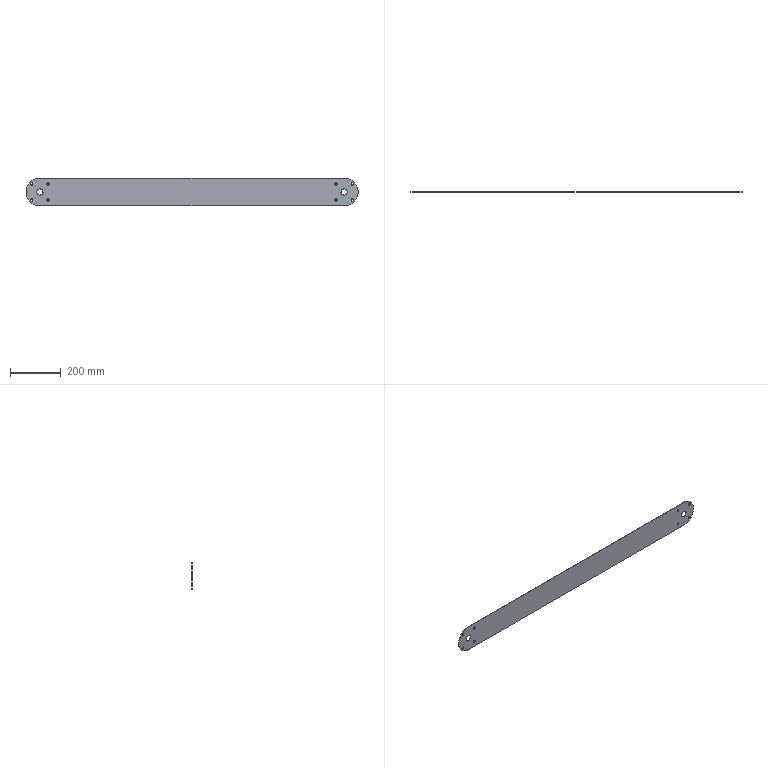Component | NX | 131_MOUNT_PLATE | 1 solid | 16 faces | volume 279787 mm3 | cylinder 12 | plane 4 | commonest cylinder face diameters 10 x8 110 x2 25 x2